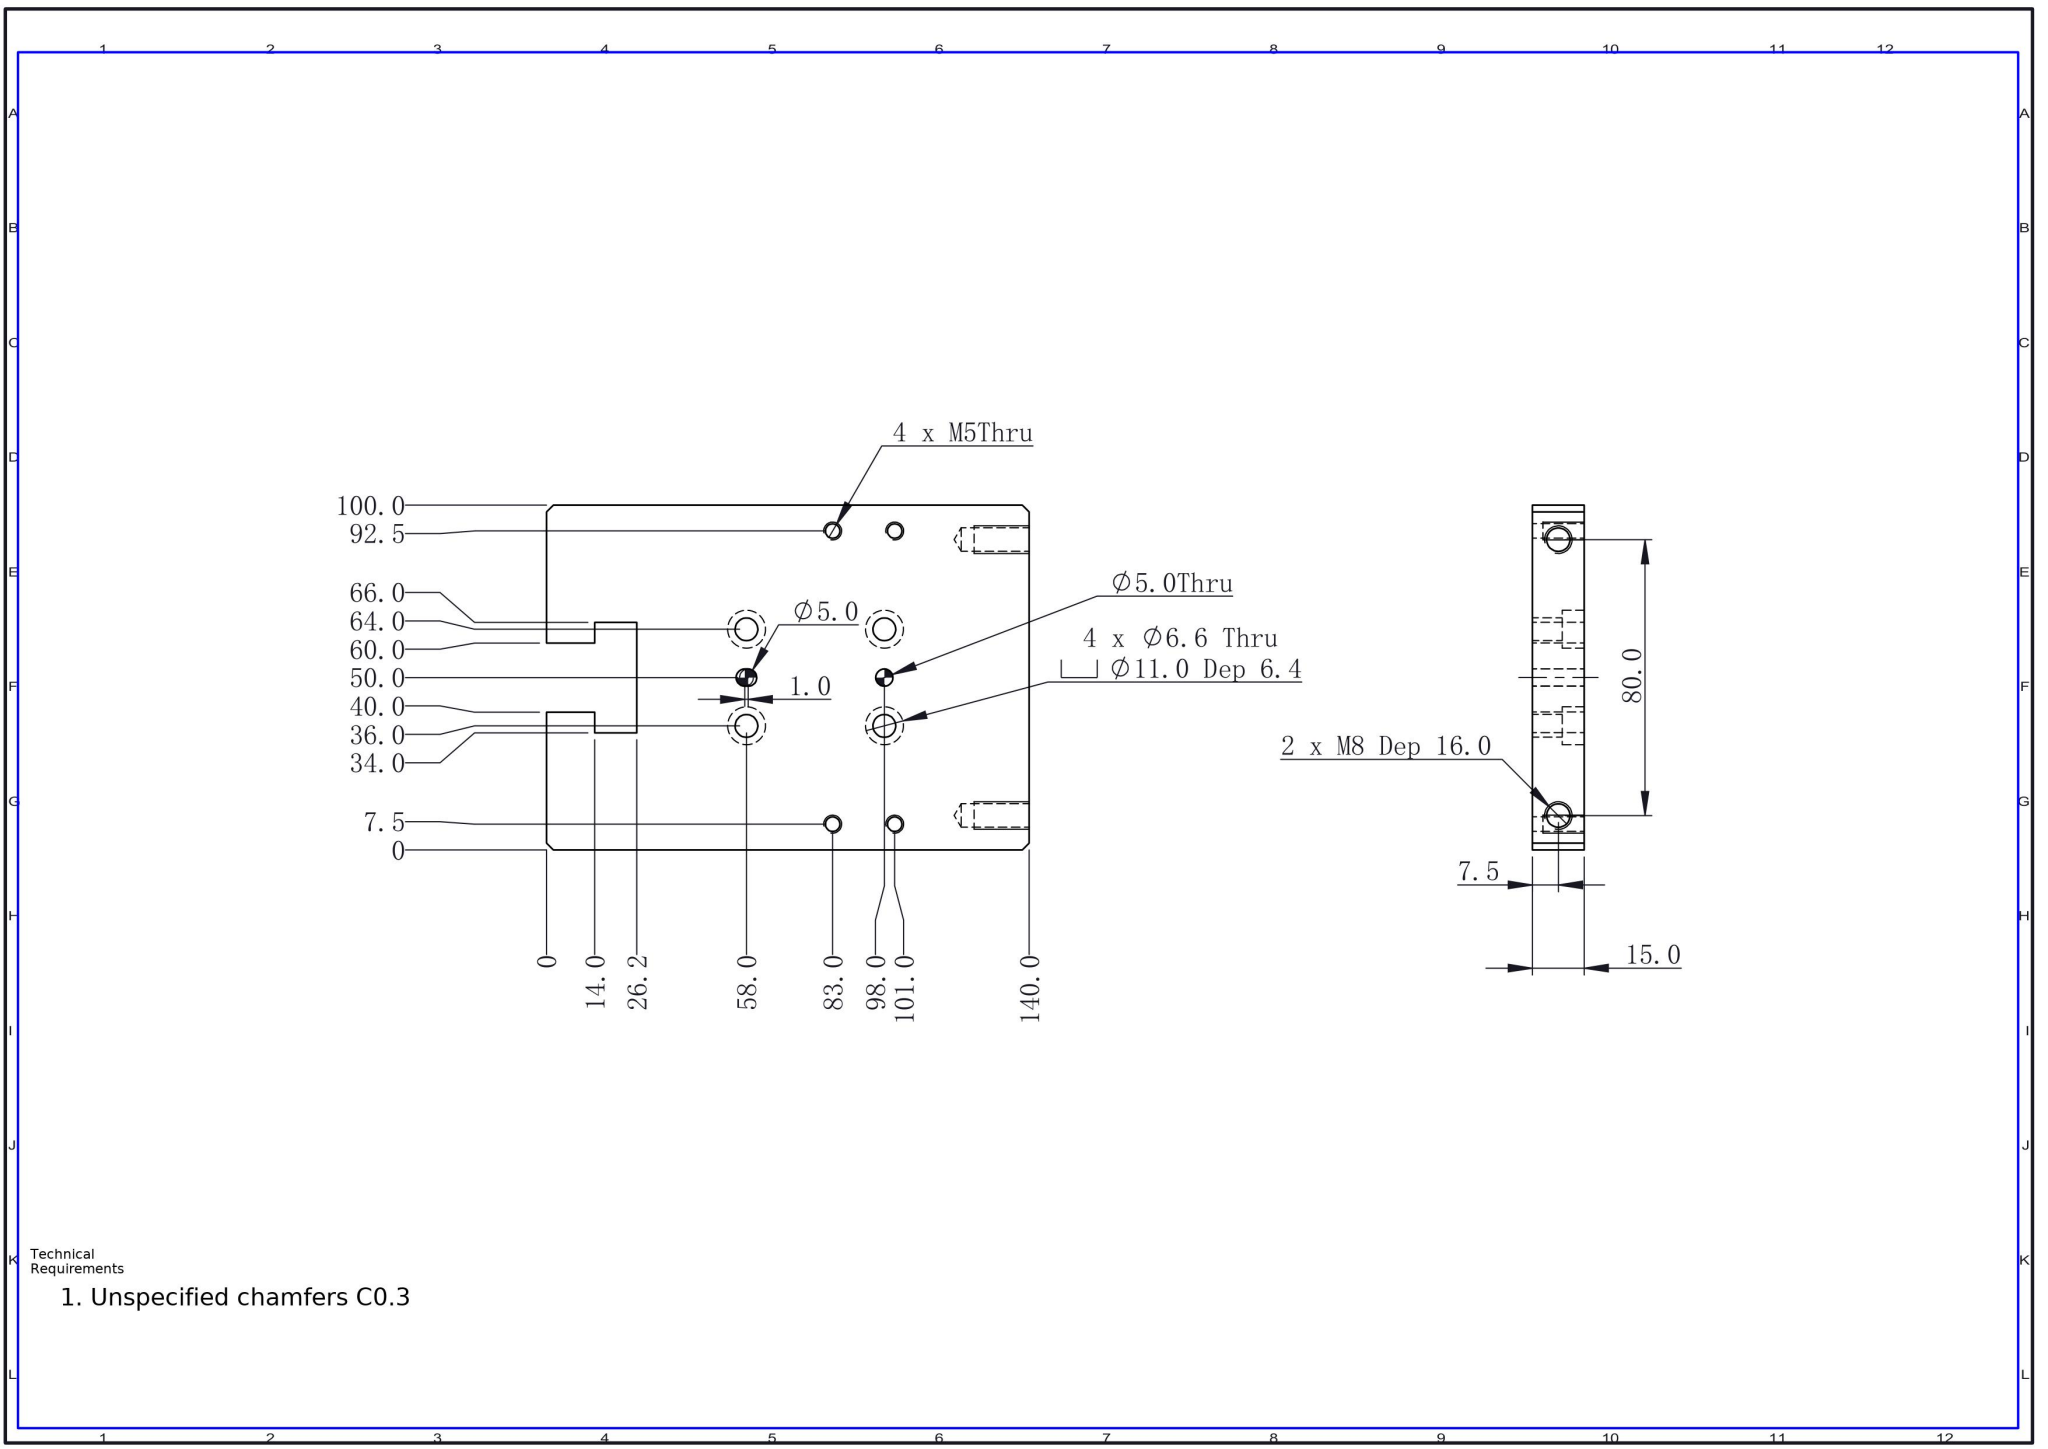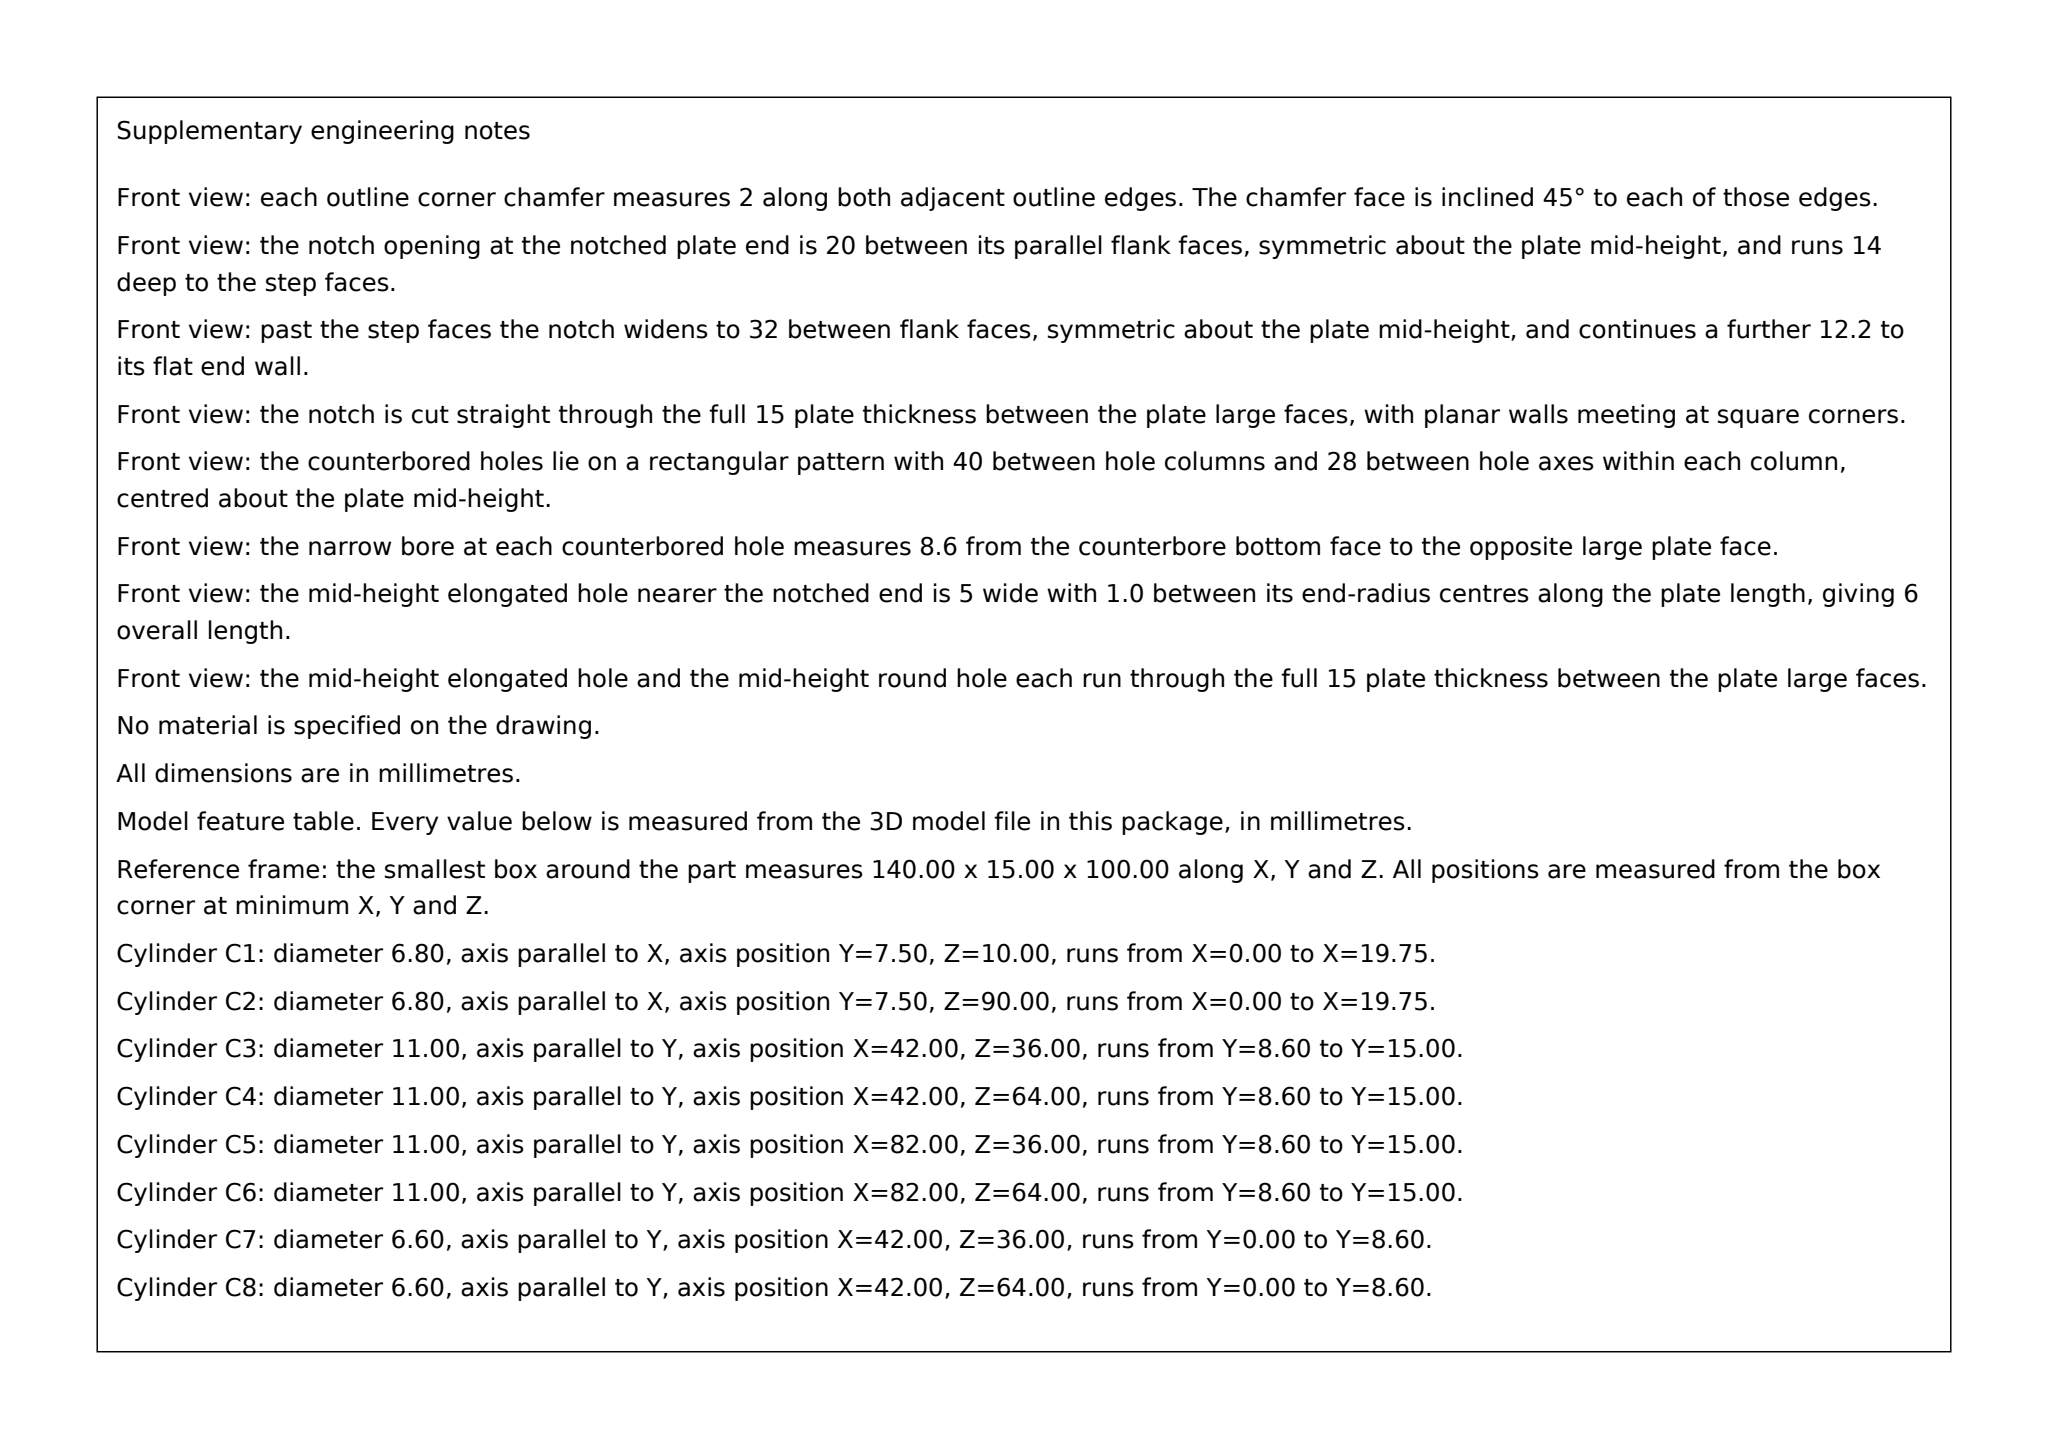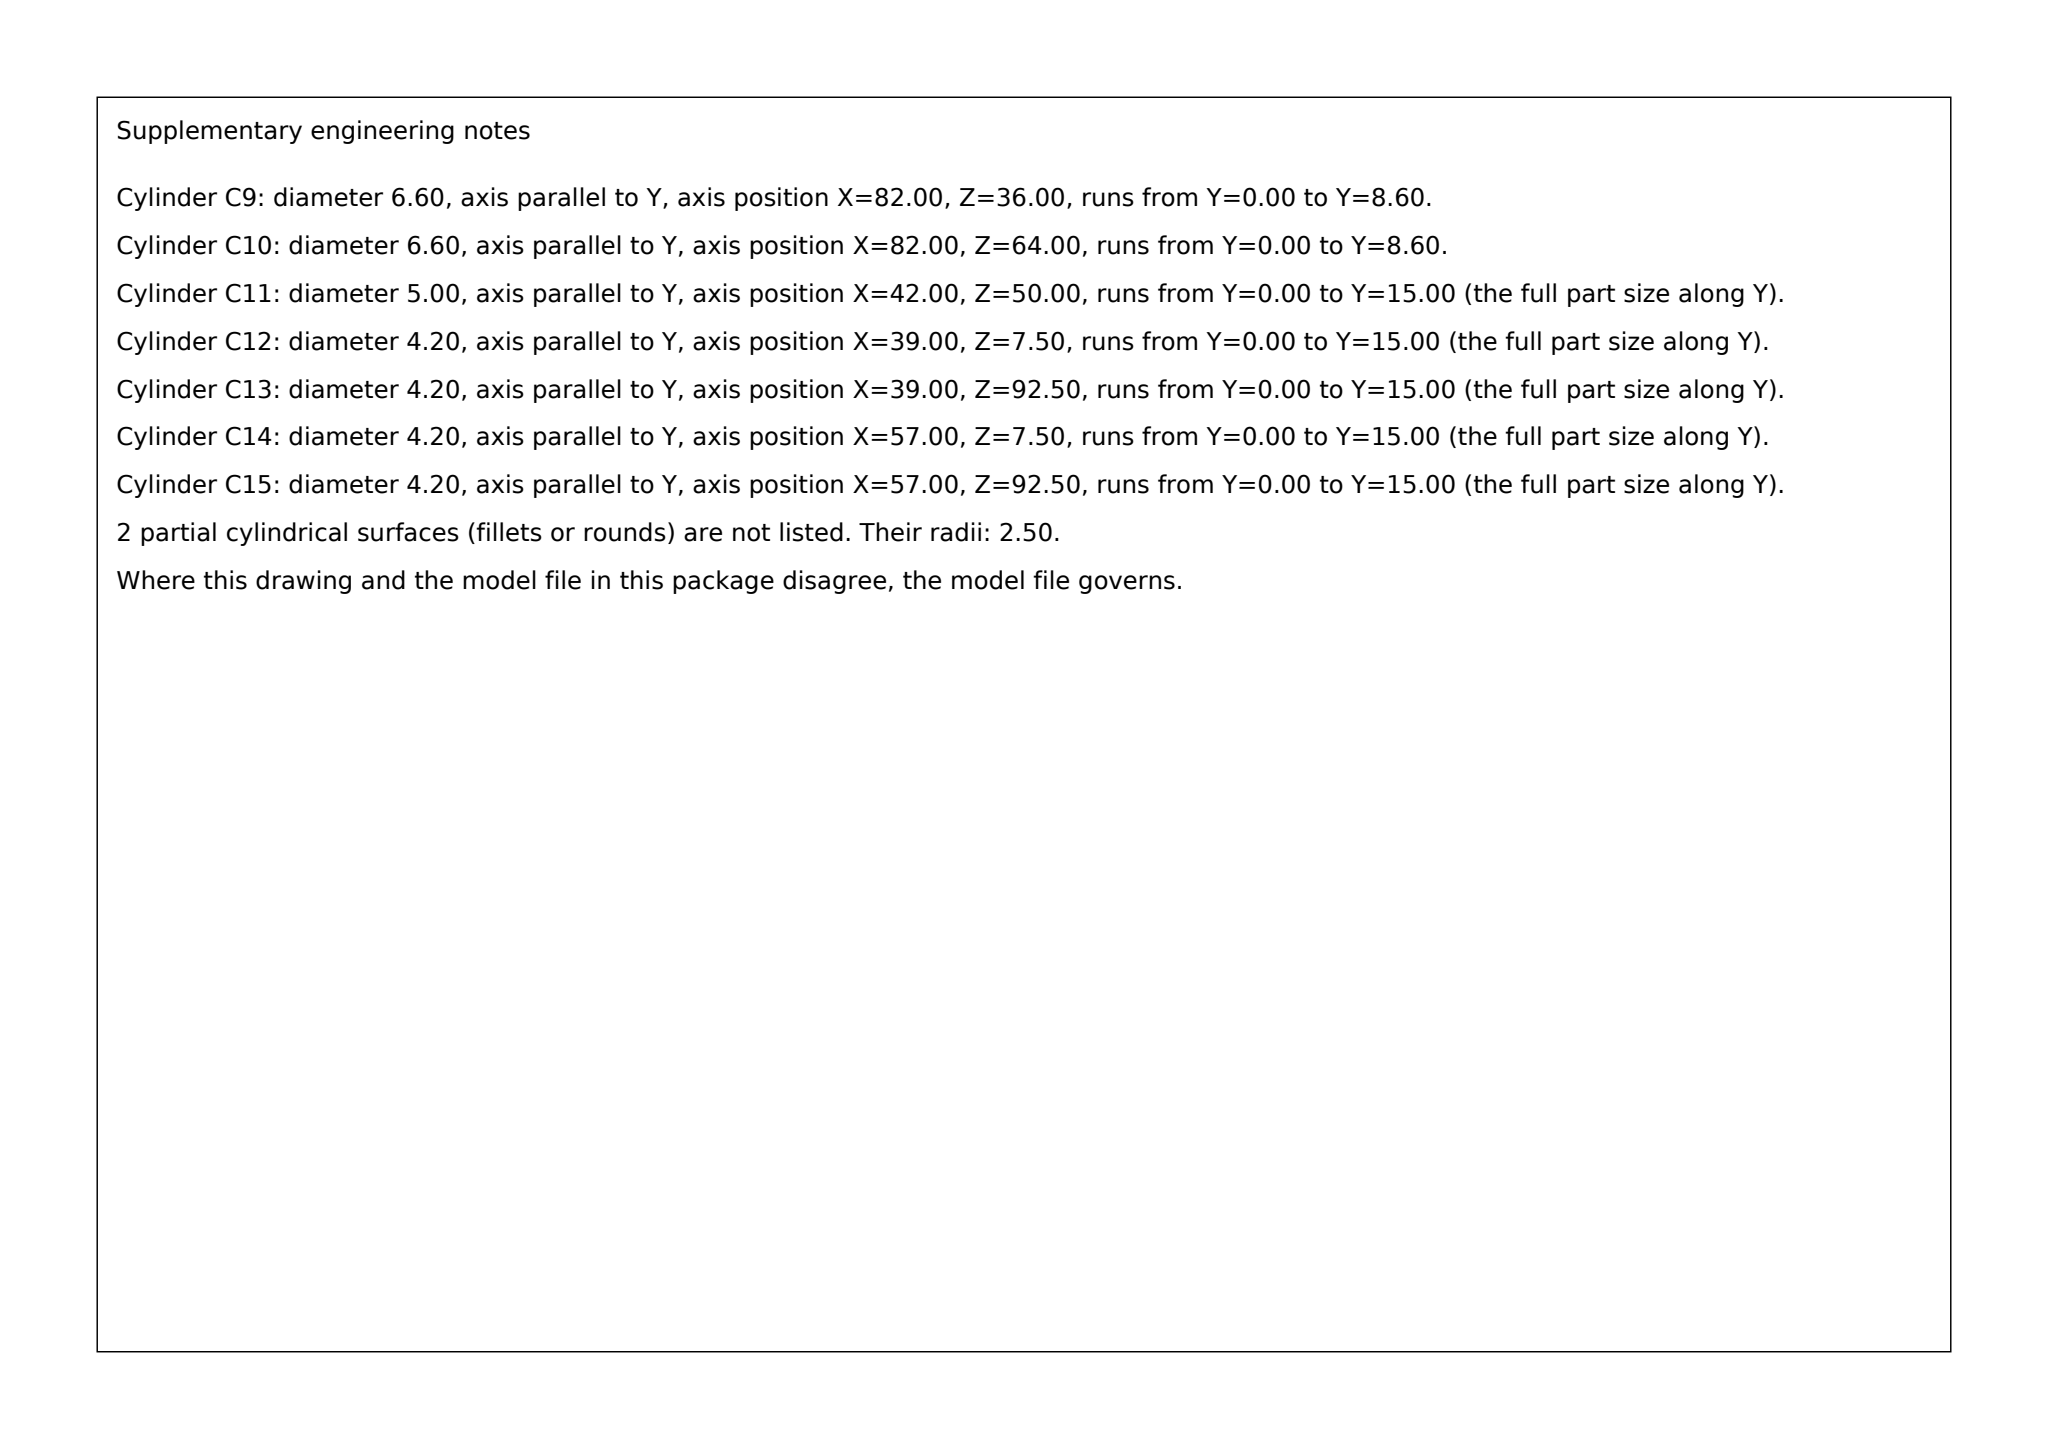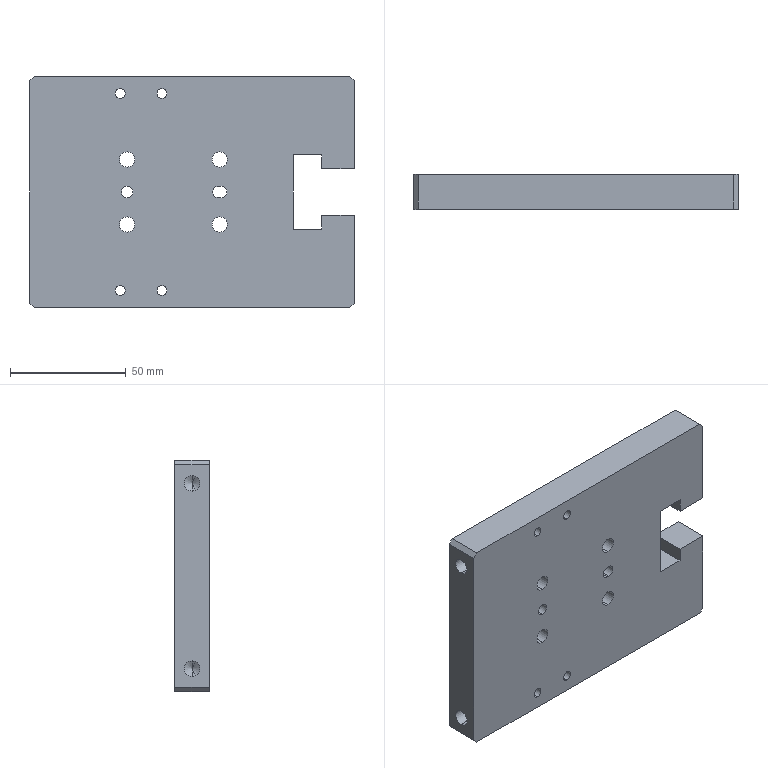Part | SolidWorks | mm | 1 solid | 60 faces | box 140 x 15 x 100 mm | volume 193235 mm3 | cylinder 32 | plane 24 | cone 4 | commonest cylinder face diameters 4.2 x8 11 x8 6.6 x8 6.8 x4 5 x4